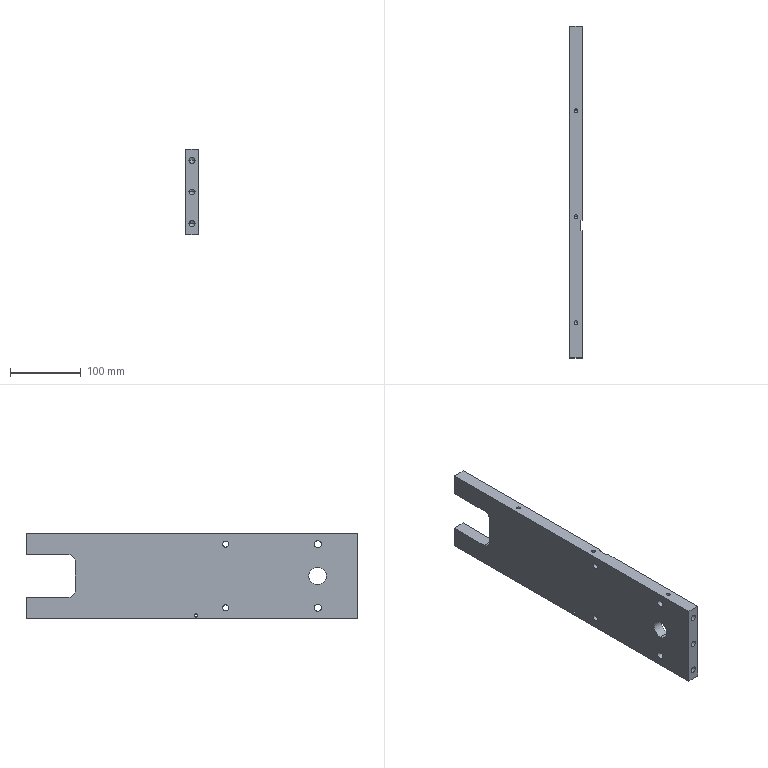Component | SolidWorks | ZL-11-06LargeUprightPlate3-1 | 1 solid | 75 faces | box 18 x 470 x 121 mm | volume 919289 mm3 | cylinder 38 | cone 22 | plane 15 | commonest cylinder face diameters 8.5 x14 5 x12 10.2 x4 44 x2 4.5 x2 25 x2 20 x2
build123d program:
from build123d import *

# Parameters (mm, degrees)
SKETCH1_2_W                 = 121
SKETCH1_2_H                 = 470
EXTRUDE1_DEPTH              = 18
F_25_0_25_DIAMETER_HOLE1_D  = 25
M12_TAPPED_HOLE1_D          = 10.2
SKETCH6_W                   = 121
SKETCH6_H                   = 15
CUT_EXTRUDE1_2_DEPTH        = 2
F_8_5_8_5_DIAMETER_HOLE1_D  = 8.5
M10_TAPPED_HOLE2_AT_2_COUNT = 2
M10_TAPPED_HOLE2_AT_2_PITCH = 45
M10_TAPPED_HOLE2_AT_3_COUNT = 2
M10_TAPPED_HOLE2_AT_3_PITCH = 45
LPATTERN1_COUNT             = 3
LPATTERN1_PITCH             = 150
SKETCH14_W                  = 60
SKETCH14_H                  = 70
CUT_EXTRUDE2_DEPTH          = 244.33
FILLET1_R                   = 10
F_4_5_4_5_DIAMETER_HOLE1_D  = 4.5
SKETCH1_R                   = 22
CUT_EXTRUDE1_DEPTH          = 3.5


with BuildPart() as part:
    # Sketch1_2 → Extrude1 (new body)
    with BuildSketch(Plane.XY):
        Rectangle(SKETCH1_2_W, SKETCH1_2_H)
    extrude(amount=EXTRUDE1_DEPTH)

    # 25.0 _25_ Diameter Hole1 (through all)
    with Locations(Plane(origin=(0, 178, 0), x_dir=(-1, 0, 0), z_dir=(0, 0, -1))):
        with Locations((0, 0)):
            Hole(F_25_0_25_DIAMETER_HOLE1_D / 2)

    # M12 Tapped Hole1 (through all)
    with Locations(Plane(origin=(45, 178, 0), x_dir=(-1, 0, 0), z_dir=(0, 0, -1))):
        with Locations((0, 0), (90, 0)):
            Hole(M12_TAPPED_HOLE1_D / 2)

    # Sketch6 → Cut-Extrude1_2 (cut)
    with BuildSketch(Plane(origin=(0, 0, 0), x_dir=(-1, 0, 0), z_dir=(0, 0, -1))):
        with Locations((0, 47.5)):
            Rectangle(SKETCH6_W, SKETCH6_H)
    extrude(amount=-CUT_EXTRUDE1_2_DEPTH, mode=Mode.SUBTRACT)

    # 8.5 _8.5_ Diameter Hole1 (through all)
    with Locations(Plane(origin=(0, 0, 2), x_dir=(-1, 0, 0), z_dir=(0, 0, -1))):
        with Locations((45, 47.5), (-45, 47.5)):
            Hole(F_8_5_8_5_DIAMETER_HOLE1_D / 2)

    # Sketch12 → M10 Tapped Hole2 (revolve, cut)
    with BuildSketch(Plane(origin=(0, 235, 9), x_dir=(0, 0, 1), z_dir=(1, 0, 0))):
        Polygon((0, 0), (0, 27.054), (4.25, 24.5), (4.25, 0), align=None)
    m10_tapped_hole2 = revolve(axis=Axis((0, 241.35, 9), (0, -1, 0)), mode=Mode.SUBTRACT)

    # M10 Tapped Hole2 at 2: M10 Tapped Hole2 ×2
    with Locations(*[(-i * M10_TAPPED_HOLE2_AT_2_PITCH, 0, 0) for i in range(1, M10_TAPPED_HOLE2_AT_2_COUNT)]):
        add(m10_tapped_hole2, mode=Mode.SUBTRACT)

    # M10 Tapped Hole2 at 3: M10 Tapped Hole2 ×2
    with Locations(*[(i * M10_TAPPED_HOLE2_AT_3_PITCH, 0, 0) for i in range(1, M10_TAPPED_HOLE2_AT_3_COUNT)]):
        add(m10_tapped_hole2, mode=Mode.SUBTRACT)

    # Sketch13 → M6 Tapped Hole1 (revolve, cut)
    with BuildSketch(Plane(origin=(-60.5, 185, 9), x_dir=(0, 0, 1), z_dir=(0, 1, 0))):
        Polygon((0, 0), (0, 11.502), (2.5, 10), (2.5, 0), align=None)
    m6_tapped_hole1 = revolve(axis=Axis((-66.85, 185, 9), (1, 0, 0)), mode=Mode.SUBTRACT)

    # LPattern1: M6 Tapped Hole1 ×3
    with Locations(*[(0, -i * LPATTERN1_PITCH, 0) for i in range(1, LPATTERN1_COUNT)]):
        add(m6_tapped_hole1, mode=Mode.SUBTRACT)

    # Mirror1: M6 Tapped Hole1 across plane
    add(m6_tapped_hole1.mirror(Plane(origin=(0, 0, 0), x_dir=(0, 0, 1), z_dir=(1, 0, 0))), mode=Mode.SUBTRACT)

    # Mirror1 copy 1 sketch → Mirror1 copy 1 (revolve, cut)
    with BuildSketch(Plane(origin=(60.5, 35, 9), x_dir=(0, 0, 1), z_dir=(0, 1, 0))):
        Polygon((0, 0), (0, -11.502), (2.5, -10), (2.5, 0), align=None)
    revolve(axis=Axis((66.85, 35, 9), (1, 0, 0)), mode=Mode.SUBTRACT)

    # Mirror1 copy 2 sketch → Mirror1 copy 2 (revolve, cut)
    with BuildSketch(Plane(origin=(60.5, -115, 9), x_dir=(0, 0, 1), z_dir=(0, 1, 0))):
        Polygon((0, 0), (0, -11.502), (2.5, -10), (2.5, 0), align=None)
    revolve(axis=Axis((66.85, -115, 9), (1, 0, 0)), mode=Mode.SUBTRACT)

    # Mirror2: M10 Tapped Hole2 across plane
    add(m10_tapped_hole2.mirror(Plane.ZX), mode=Mode.SUBTRACT)

    # Mirror2 copy 1 sketch → Mirror2 copy 1 (revolve, cut)
    with BuildSketch(Plane(origin=(-45, -235, 9), x_dir=(0, 0, 1), z_dir=(1, 0, 0))):
        Polygon((0, 0), (0, -27.054), (4.25, -24.5), (4.25, 0), align=None)
    revolve(axis=Axis((-45, -241.35, 9), (0, -1, 0)), mode=Mode.SUBTRACT)

    # Mirror2 copy 2 sketch → Mirror2 copy 2 (revolve, cut)
    with BuildSketch(Plane(origin=(45, -235, 9), x_dir=(0, 0, 1), z_dir=(1, 0, 0))):
        Polygon((0, 0), (0, -27.054), (4.25, -24.5), (4.25, 0), align=None)
    revolve(axis=Axis((45, -241.35, 9), (0, -1, 0)), mode=Mode.SUBTRACT)

    # Sketch14 → Cut-Extrude2 (cut, through all)
    with BuildSketch(Plane(origin=(0, 0, 0), x_dir=(-1, 0, 0), z_dir=(0, 0, -1))):
        with Locations((0, -200)):
            Rectangle(SKETCH14_W, SKETCH14_H)
    extrude(amount=-CUT_EXTRUDE2_DEPTH, mode=Mode.SUBTRACT)

    # Fillet1
    fillet1_edges = [part.edges().sort_by_distance(p)[0] for p in [
        (30, -165, 9),
        (-30, -165, 9),
    ]]
    fillet(fillet1_edges, radius=FILLET1_R)

    # 4.5 _4.5_ Diameter Hole1 (through all)
    with Locations(Plane(origin=(56, 6, 0), x_dir=(-1, 0, 0), z_dir=(0, 0, -1))):
        with Locations((0, 0)):
            Hole(F_4_5_4_5_DIAMETER_HOLE1_D / 2)

    # Sketch1 → Cut-Extrude1 (cut, symmetric)
    with BuildSketch(Plane.XY):
        with Locations((0, 178)):
            Circle(SKETCH1_R)
    extrude(amount=CUT_EXTRUDE1_DEPTH, both=True, mode=Mode.SUBTRACT)


solid = part.part

# Placed as in the assembly
solid = solid.moved(Location((75.552, 289.22, 0), (180, -90, 0)))